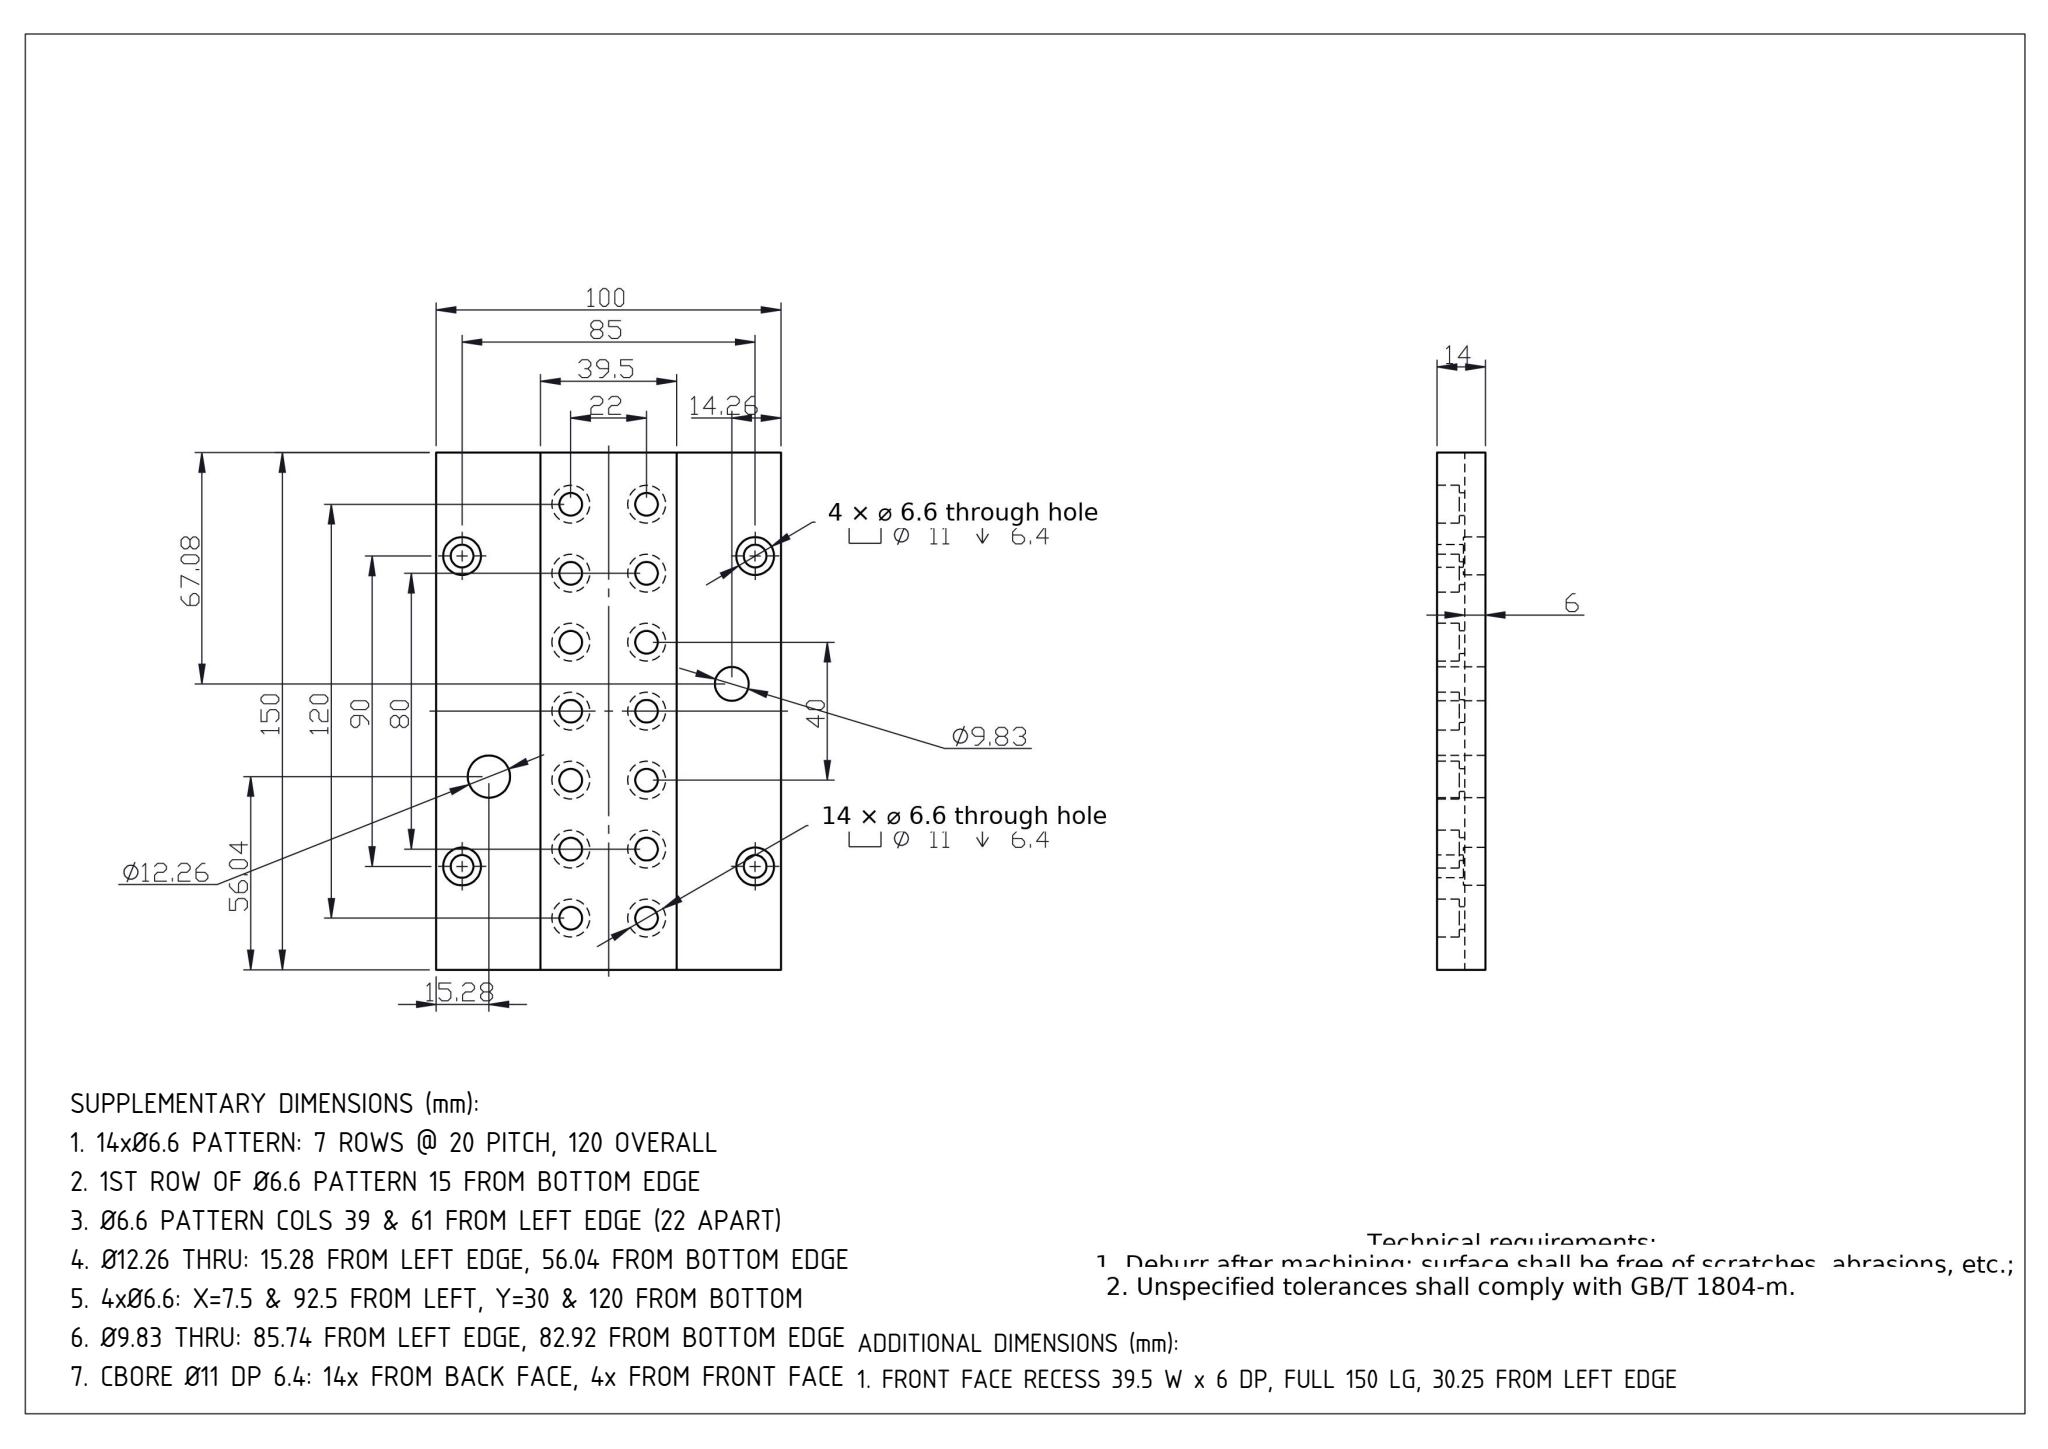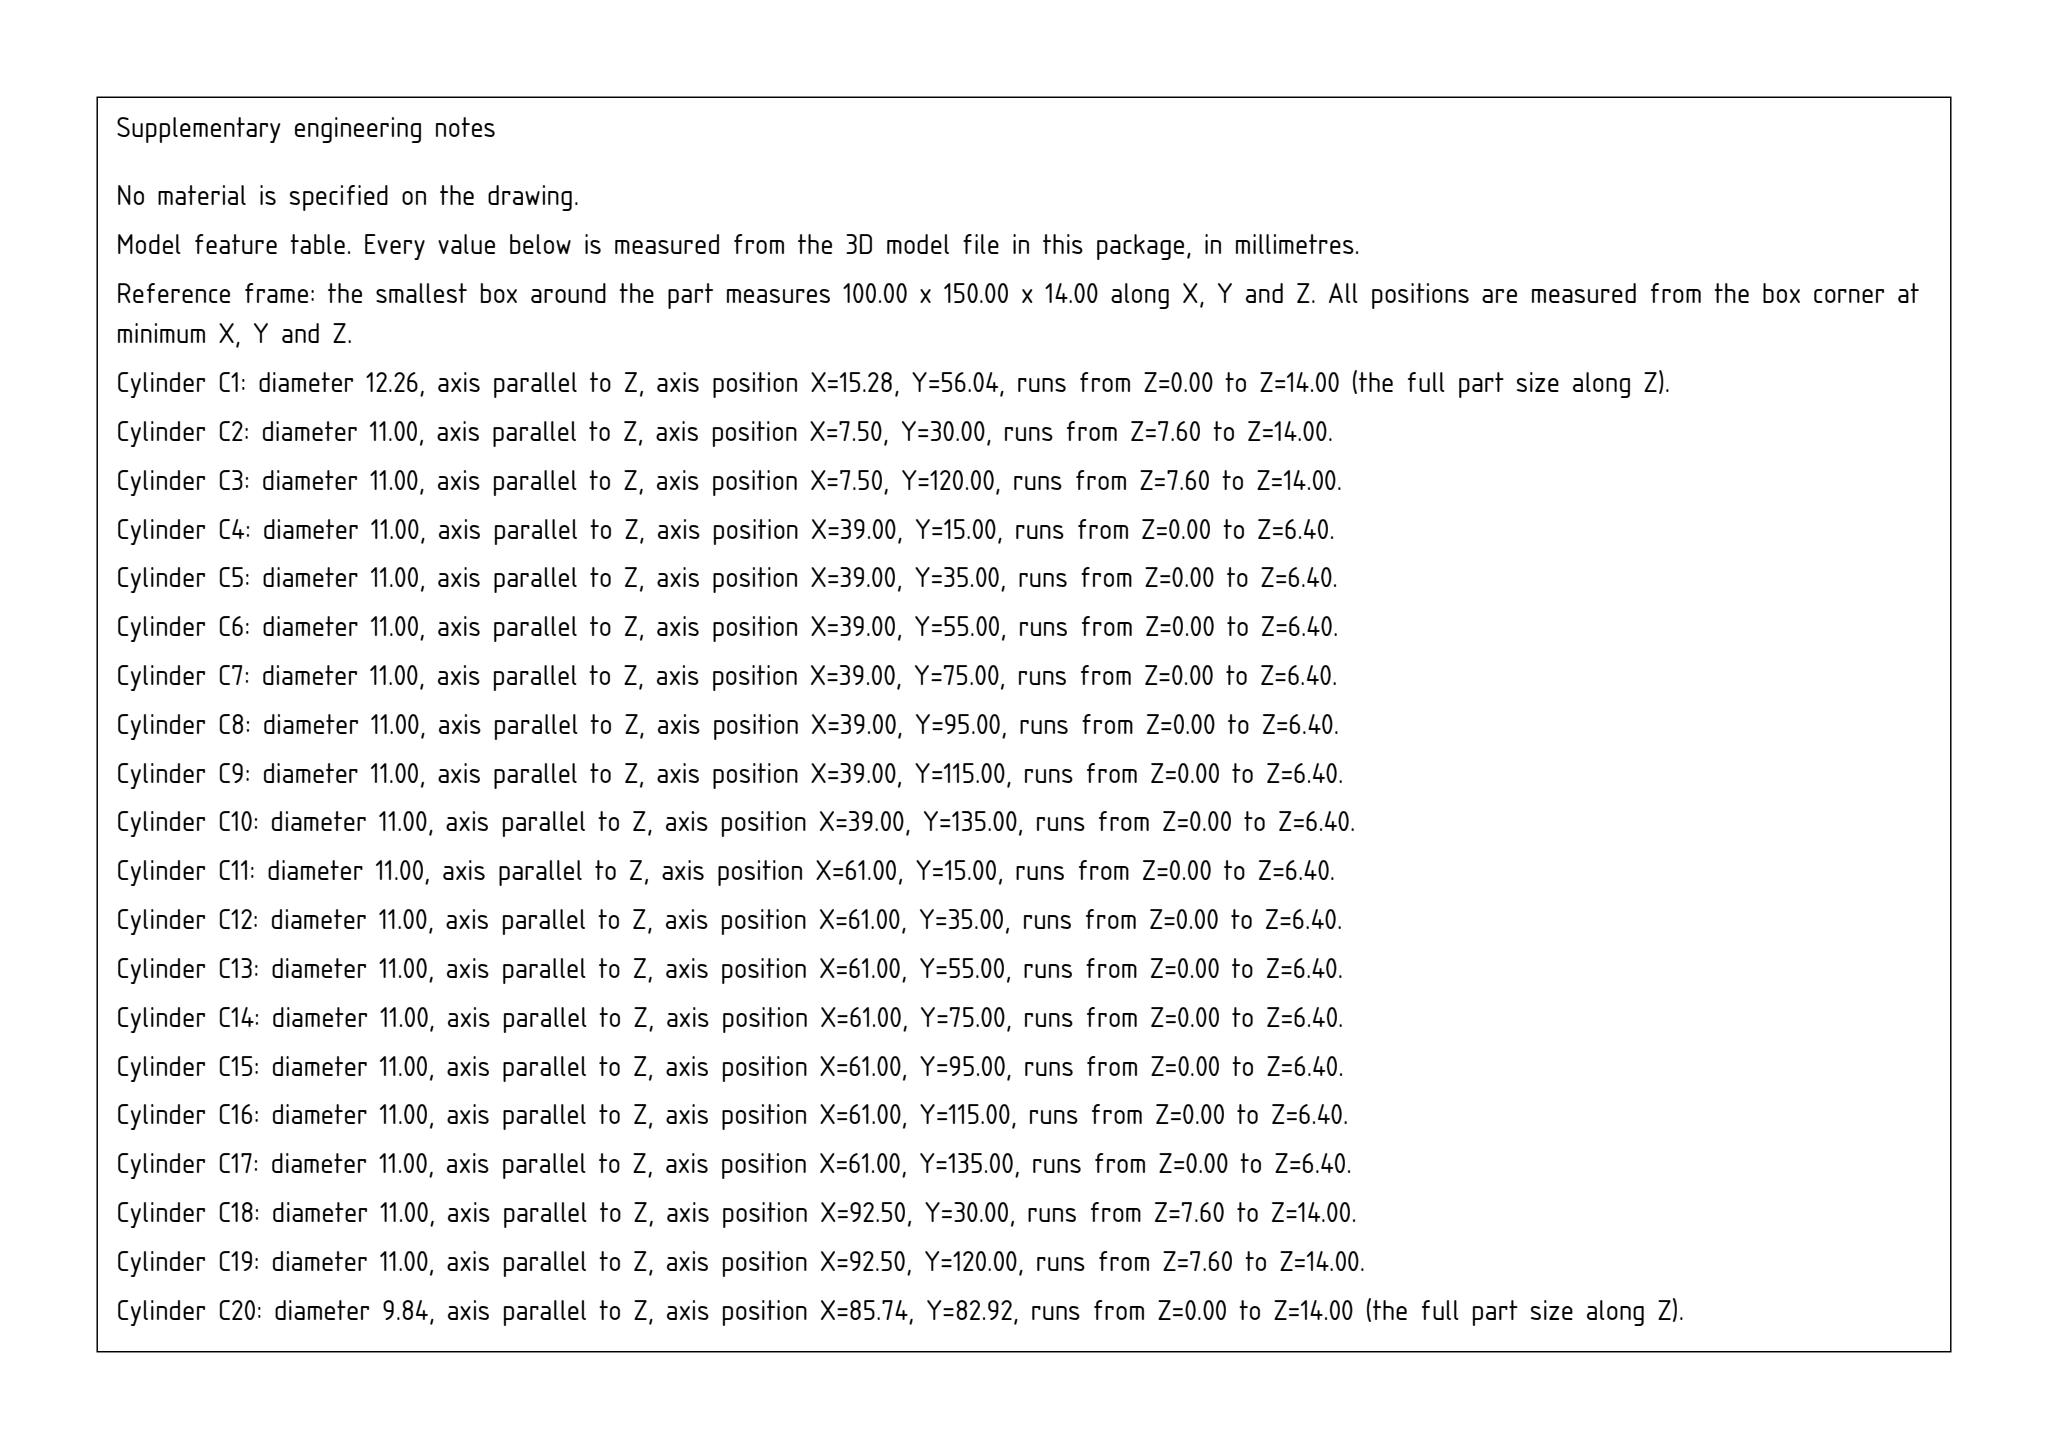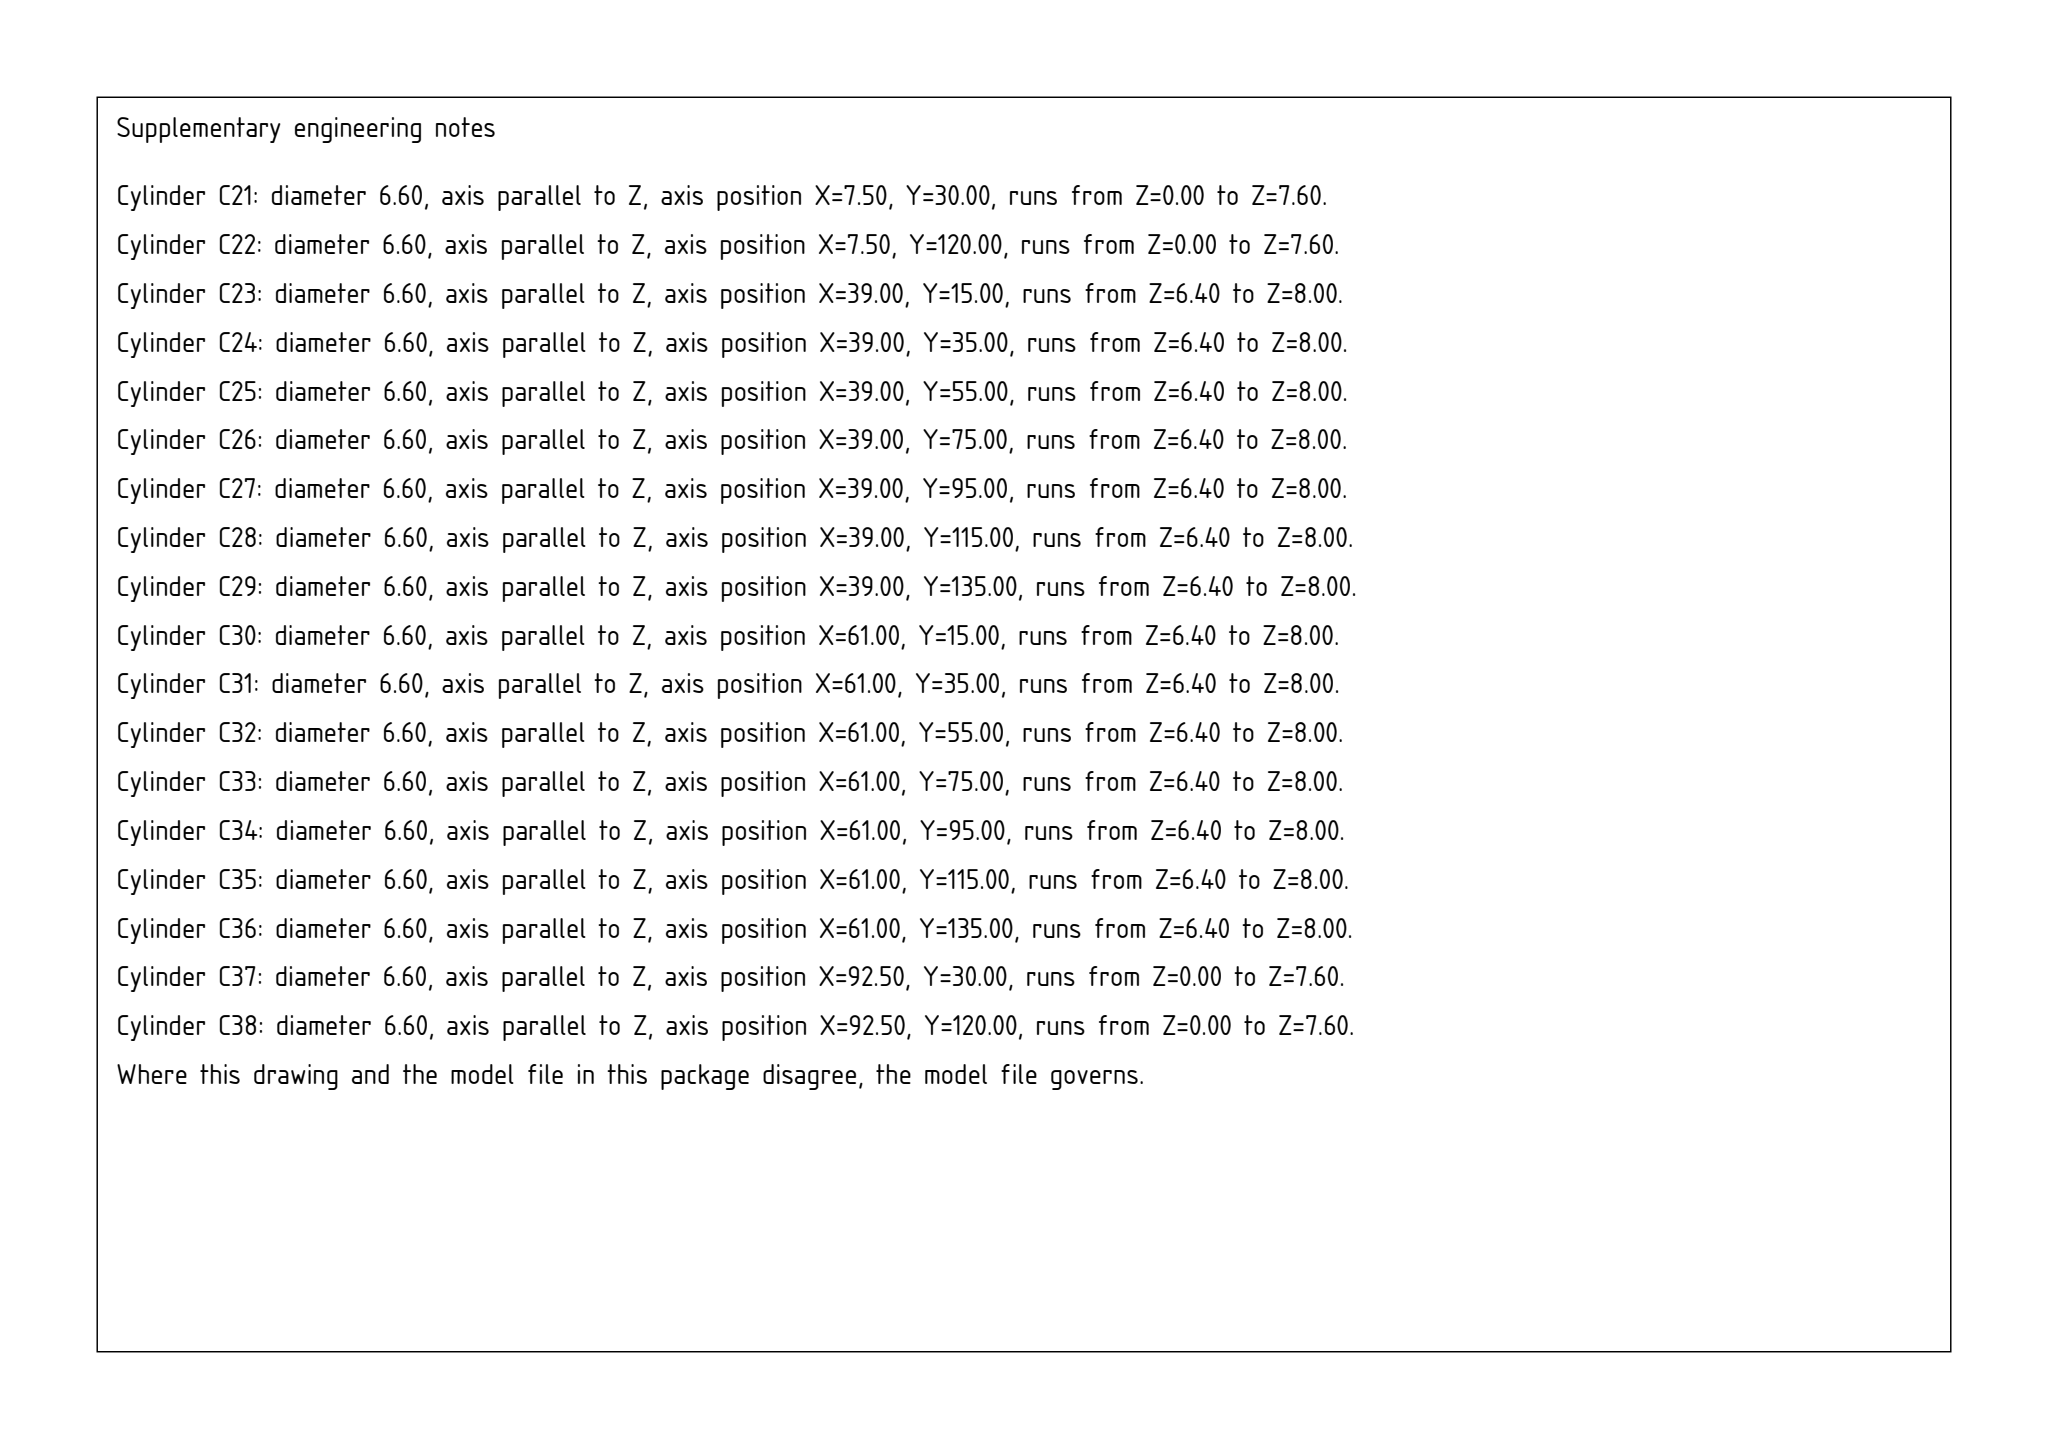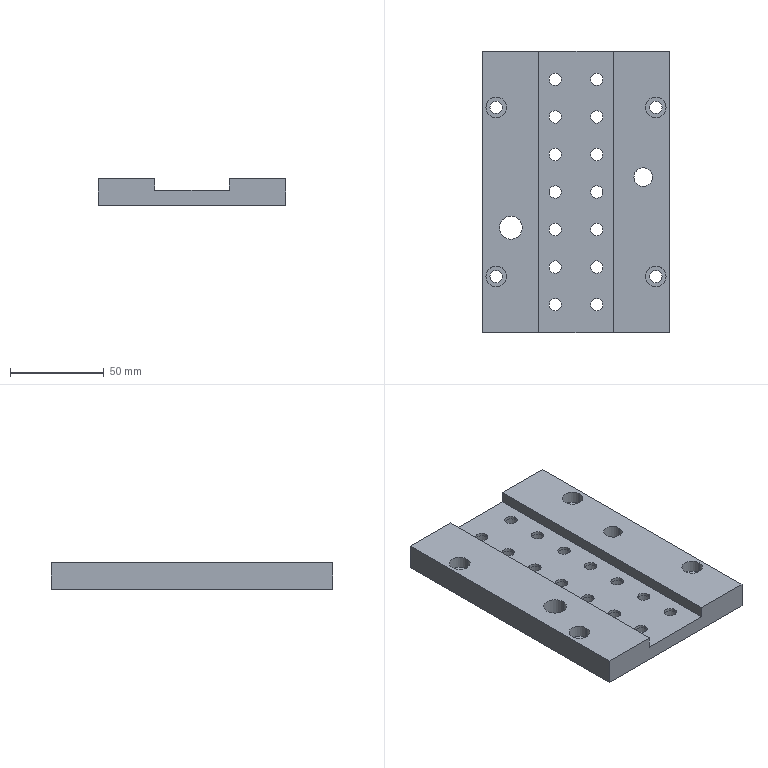Part | SolidWorks | mm | 1 solid | 104 faces | box 100 x 150 x 14 mm | volume 158980 mm3 | cylinder 76 | plane 28 | commonest cylinder face diameters 11 x36 6.6 x36 9.833 x2 12.26 x2
build123d program:
from build123d import *

# Parameters (mm, degrees)
SKETCH1_W                                       = 100
SKETCH1_H                                       = 150
BOSS_EXTRUDE1_DEPTH                             = 14
SKETCH2_W                                       = 39.5
SKETCH2_H                                       = 150
CUT_EXTRUDE1_DEPTH                              = 6
M6_HEX_SOCKET_HEAD_CAP_SCREW_CBORE1_D           = 6.6
M6_HEX_SOCKET_HEAD_CAP_SCREW_CBORE1_CBORE_D     = 11
M6_HEX_SOCKET_HEAD_CAP_SCREW_CBORE1_CBORE_DEPTH = 6.4
M6_HEX_SOCKET_HEAD_CAP_SCREW_CBORE2_D           = 6.6
M6_HEX_SOCKET_HEAD_CAP_SCREW_CBORE2_CBORE_D     = 11
M6_HEX_SOCKET_HEAD_CAP_SCREW_CBORE2_CBORE_DEPTH = 6.4
SKETCH7_R                                       = 4.916
SKETCH7_R_2                                     = 6.13
CUT_EXTRUDE2_DEPTH                              = 61


with BuildPart() as part:
    # Sketch1 → Boss-Extrude1 (new body)
    with BuildSketch(Plane.XY):
        with Locations((50, -75)):
            Rectangle(SKETCH1_W, SKETCH1_H)
    extrude(amount=BOSS_EXTRUDE1_DEPTH)

    # Sketch2 → Cut-Extrude1 (cut)
    with BuildSketch(Plane.XY.offset(14)):
        with Locations((50, -75)):
            Rectangle(SKETCH2_W, SKETCH2_H)
    extrude(amount=-CUT_EXTRUDE1_DEPTH, mode=Mode.SUBTRACT)

    # M6 Hex Socket Head Cap Screw CBORE1 (through all)
    with Locations(Plane(origin=(-28.941, 14.88, 0), x_dir=(1, 0, 0), z_dir=(0, 0, -1))):
        with Locations((67.941, 29.88), (89.941, 29.88), (89.941, 69.88), (67.941, 69.88), (67.941, 109.88), (89.941, 109.88), (89.941, 149.88), (67.941, 149.88), (67.941, 49.88), (89.941, 49.88), (89.941, 89.88), (67.941, 89.88), (67.941, 129.88), (89.941, 129.88)):
            CounterBoreHole(M6_HEX_SOCKET_HEAD_CAP_SCREW_CBORE1_D / 2, M6_HEX_SOCKET_HEAD_CAP_SCREW_CBORE1_CBORE_D / 2, M6_HEX_SOCKET_HEAD_CAP_SCREW_CBORE1_CBORE_DEPTH)

    # M6 Hex Socket Head Cap Screw CBORE2 (through all)
    with Locations(Plane.XY.offset(14)):
        with Locations((7.5, -30), (7.5, -120), (92.5, -30), (92.5, -120)):
            CounterBoreHole(M6_HEX_SOCKET_HEAD_CAP_SCREW_CBORE2_D / 2, M6_HEX_SOCKET_HEAD_CAP_SCREW_CBORE2_CBORE_D / 2, M6_HEX_SOCKET_HEAD_CAP_SCREW_CBORE2_CBORE_DEPTH)

    # Sketch7 → Cut-Extrude2 (cut)
    with BuildSketch(Plane(origin=(0, 0, 0), x_dir=(-1, 0, 0), z_dir=(0, 0, -1))):
        with Locations((-85.741, -67.082)):
            Circle(SKETCH7_R)
        with Locations((-15.276, -93.96)):
            Circle(SKETCH7_R_2)
    extrude(amount=-CUT_EXTRUDE2_DEPTH, mode=Mode.SUBTRACT)


solid = part.part